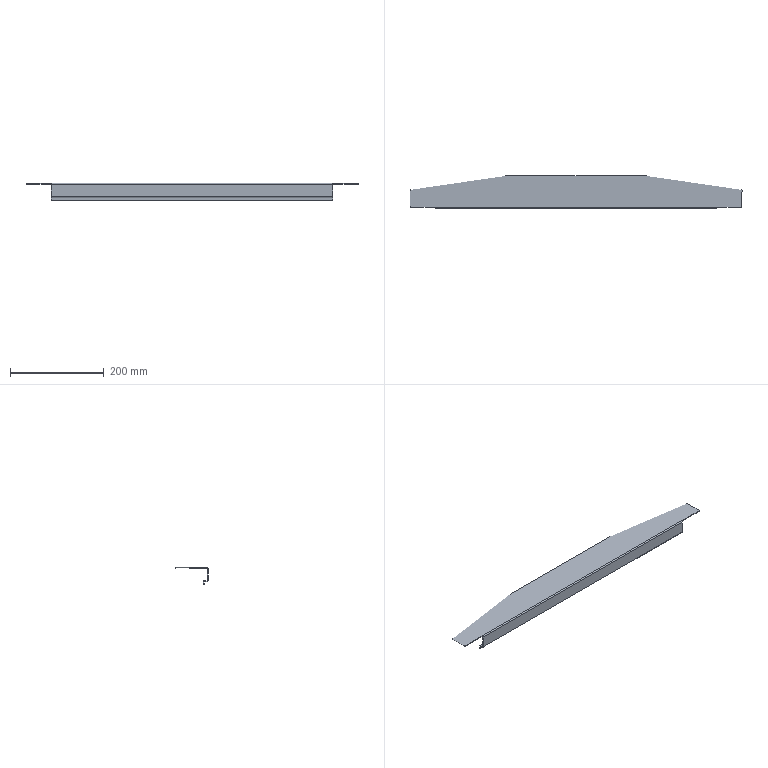Component | SolidWorks | TopCover01100-2_TopCoverPlug01100-1 | 1 solid | 49 faces | volume 100709 mm3 | plane 43 | cylinder 6 | commonest cylinder face diameters 4.473 x3 1.473 x3